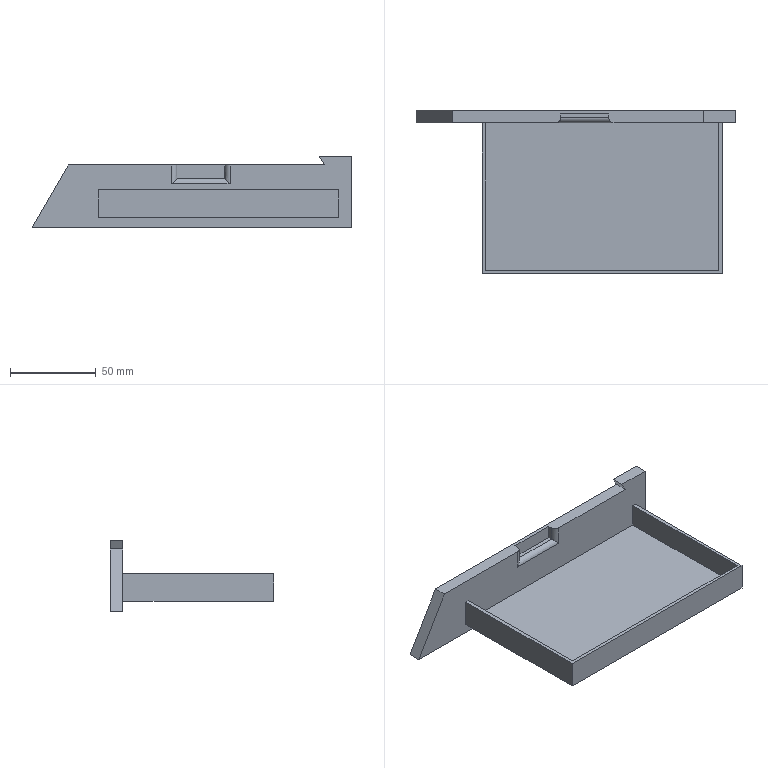Component | NX | DRAWER_2 | 1 solid | 24 faces | volume 79643 mm3 | plane 21 | cylinder 3 | commonest cylinder face diameters 6 x3